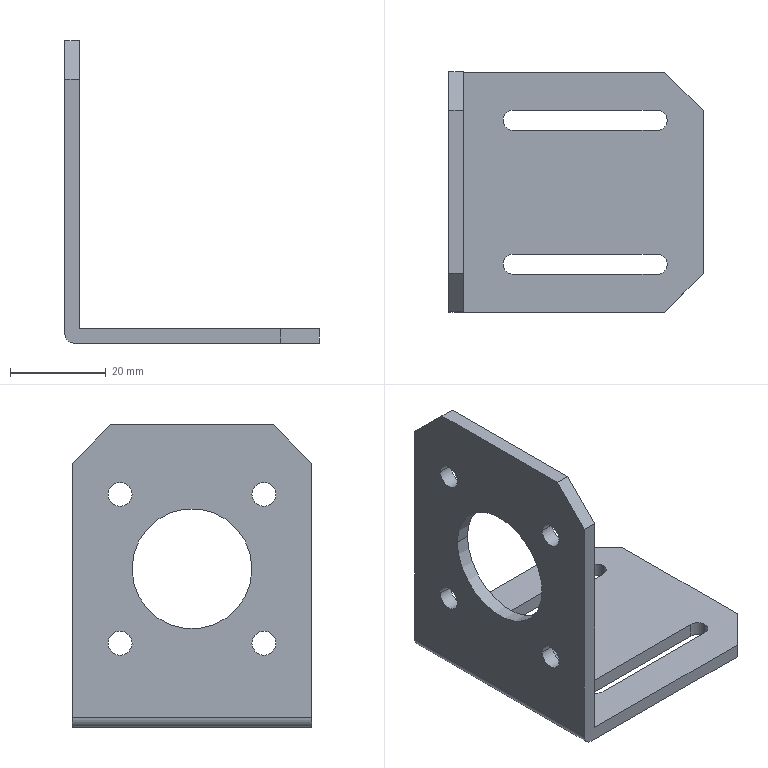Component | SolidWorks | Mount-3 | 1 solid | 33 faces | box 53 x 50 x 63 mm | volume 13976 mm3 | cylinder 17 | plane 16 | commonest cylinder face diameters 5 x8 4.2 x6 25 x2 4 x1
STEP:
#1=COLOUR_RGB('',0.7922,0.8196,0.9333);
#2=FILL_AREA_STYLE_COLOUR('',#1);
#3=FILL_AREA_STYLE('',(#2));
#4=SURFACE_STYLE_FILL_AREA(#3);
#5=SURFACE_SIDE_STYLE('',(#4));
#6=SURFACE_STYLE_USAGE(.BOTH.,#5);
#7=PRESENTATION_STYLE_ASSIGNMENT((#6));
#8=CARTESIAN_POINT('',(-2.678,-2.594,0.1575));
#9=VERTEX_POINT('',#8);
#10=CARTESIAN_POINT('',(-2.595,-2.677,0.1575));
#11=VERTEX_POINT('',#10);
#12=CARTESIAN_POINT('',(-2.678,-2.677,0.1575));
#13=DIRECTION('',(-0.,0.,-1.));
#14=DIRECTION('',(1.,0.,0.));
#15=AXIS2_PLACEMENT_3D('',#12,#13,#14);
#16=CIRCLE('',#15,0.08268);
#17=EDGE_CURVE('',#9,#11,#16,.T.);
#18=ORIENTED_EDGE('',*,*,#17,.T.);
#19=CARTESIAN_POINT('',(-2.595,-2.677,0.2756));
#20=VERTEX_POINT('',#19);
#21=CARTESIAN_POINT('',(-2.595,-2.677,0.1575));
#22=DIRECTION('',(0.,-0.,1.));
#23=VECTOR('',#22,39.37);
#24=LINE('',#21,#23);
#25=EDGE_CURVE('',#11,#20,#24,.T.);
#26=ORIENTED_EDGE('',*,*,#25,.T.);
#27=CARTESIAN_POINT('',(-2.678,-2.594,0.2756));
#28=VERTEX_POINT('',#27);
#29=CARTESIAN_POINT('',(-2.678,-2.677,0.2756));
#30=DIRECTION('',(-0.,0.,-1.));
#31=DIRECTION('',(1.,0.,0.));
#32=AXIS2_PLACEMENT_3D('',#29,#30,#31);
#33=CIRCLE('',#32,0.08268);
#34=EDGE_CURVE('',#28,#20,#33,.T.);
#35=ORIENTED_EDGE('',*,*,#34,.F.);
#36=CARTESIAN_POINT('',(-2.678,-2.594,0.1575));
#37=DIRECTION('',(0.,-0.,1.));
#38=VECTOR('',#37,39.37);
#39=LINE('',#36,#38);
#40=EDGE_CURVE('',#9,#28,#39,.T.);
#41=ORIENTED_EDGE('',*,*,#40,.F.);
#42=EDGE_LOOP('',(#18,#26,#35,#41));
#43=FACE_OUTER_BOUND('',#42,.T.);
#44=CARTESIAN_POINT('',(-2.678,-2.677,0.1575));
#45=DIRECTION('',(0.,-0.,1.));
#46=DIRECTION('',(1.,0.,0.));
#47=AXIS2_PLACEMENT_3D('',#44,#45,#46);
#48=CYLINDRICAL_SURFACE('',#47,0.08268);
#49=ADVANCED_FACE('',(#43),#48,.F.);
#50=CARTESIAN_POINT('',(-2.678,-3.776,0.1575));
#51=VERTEX_POINT('',#50);
#52=CARTESIAN_POINT('',(-2.595,-3.858,0.1575));
#53=VERTEX_POINT('',#52);
#54=CARTESIAN_POINT('',(-2.678,-3.858,0.1575));
#55=DIRECTION('',(-0.,0.,-1.));
#56=DIRECTION('',(-1.,0.,0.));
#57=AXIS2_PLACEMENT_3D('',#54,#55,#56);
#58=CIRCLE('',#57,0.08268);
#59=EDGE_CURVE('',#51,#53,#58,.T.);
#60=ORIENTED_EDGE('',*,*,#59,.T.);
#61=CARTESIAN_POINT('',(-2.595,-3.858,0.2756));
#62=VERTEX_POINT('',#61);
#63=CARTESIAN_POINT('',(-2.595,-3.858,0.1575));
#64=DIRECTION('',(0.,-0.,1.));
#65=VECTOR('',#64,39.37);
#66=LINE('',#63,#65);
#67=EDGE_CURVE('',#53,#62,#66,.T.);
#68=ORIENTED_EDGE('',*,*,#67,.T.);
#69=CARTESIAN_POINT('',(-2.678,-3.776,0.2756));
#70=VERTEX_POINT('',#69);
#71=CARTESIAN_POINT('',(-2.678,-3.858,0.2756));
#72=DIRECTION('',(-0.,0.,-1.));
#73=DIRECTION('',(-1.,0.,0.));
#74=AXIS2_PLACEMENT_3D('',#71,#72,#73);
#75=CIRCLE('',#74,0.08268);
#76=EDGE_CURVE('',#70,#62,#75,.T.);
#77=ORIENTED_EDGE('',*,*,#76,.F.);
#78=CARTESIAN_POINT('',(-2.678,-3.776,0.1575));
#79=DIRECTION('',(0.,-0.,1.));
#80=VECTOR('',#79,39.37);
#81=LINE('',#78,#80);
#82=EDGE_CURVE('',#51,#70,#81,.T.);
#83=ORIENTED_EDGE('',*,*,#82,.F.);
#84=EDGE_LOOP('',(#60,#68,#77,#83));
#85=FACE_OUTER_BOUND('',#84,.T.);
#86=CARTESIAN_POINT('',(-2.678,-3.858,0.1575));
#87=DIRECTION('',(0.,-0.,1.));
#88=DIRECTION('',(1.,0.,0.));
#89=AXIS2_PLACEMENT_3D('',#86,#87,#88);
#90=CYLINDRICAL_SURFACE('',#89,0.08268);
#91=ADVANCED_FACE('',(#85),#90,.F.);
#92=CARTESIAN_POINT('',(-4.268,-3.76,1.457));
#93=VERTEX_POINT('',#92);
#94=CARTESIAN_POINT('',(-4.268,-2.776,1.457));
#95=VERTEX_POINT('',#94);
#96=CARTESIAN_POINT('',(-4.268,-3.268,1.457));
#97=DIRECTION('',(1.,0.,-0.));
#98=DIRECTION('',(-0.,1.,0.));
#99=AXIS2_PLACEMENT_3D('',#96,#97,#98);
#100=CIRCLE('',#99,0.4921);
#101=EDGE_CURVE('',#93,#95,#100,.T.);
#102=ORIENTED_EDGE('',*,*,#101,.T.);
#103=CARTESIAN_POINT('',(-4.387,-2.776,1.457));
#104=VERTEX_POINT('',#103);
#105=CARTESIAN_POINT('',(-4.268,-2.776,1.457));
#106=DIRECTION('',(-1.,-0.,0.));
#107=VECTOR('',#106,39.37);
#108=LINE('',#105,#107);
#109=EDGE_CURVE('',#95,#104,#108,.T.);
#110=ORIENTED_EDGE('',*,*,#109,.T.);
#111=CARTESIAN_POINT('',(-4.387,-3.76,1.457));
#112=VERTEX_POINT('',#111);
#113=CARTESIAN_POINT('',(-4.387,-3.268,1.457));
#114=DIRECTION('',(1.,0.,-0.));
#115=DIRECTION('',(-0.,1.,0.));
#116=AXIS2_PLACEMENT_3D('',#113,#114,#115);
#117=CIRCLE('',#116,0.4921);
#118=EDGE_CURVE('',#112,#104,#117,.T.);
#119=ORIENTED_EDGE('',*,*,#118,.F.);
#120=CARTESIAN_POINT('',(-4.268,-3.76,1.457));
#121=DIRECTION('',(-1.,-0.,0.));
#122=VECTOR('',#121,39.37);
#123=LINE('',#120,#122);
#124=EDGE_CURVE('',#93,#112,#123,.T.);
#125=ORIENTED_EDGE('',*,*,#124,.F.);
#126=EDGE_LOOP('',(#102,#110,#119,#125));
#127=FACE_OUTER_BOUND('',#126,.T.);
#128=CARTESIAN_POINT('',(-4.268,-3.268,1.457));
#129=DIRECTION('',(-1.,-0.,0.));
#130=DIRECTION('',(0.,-1.,0.));
#131=AXIS2_PLACEMENT_3D('',#128,#129,#130);
#132=CYLINDRICAL_SURFACE('',#131,0.4921);
#133=ADVANCED_FACE('',(#127),#132,.F.);
#134=CARTESIAN_POINT('',(-4.268,-3.957,2.067));
#135=VERTEX_POINT('',#134);
#136=CARTESIAN_POINT('',(-4.268,-3.76,2.067));
#137=VERTEX_POINT('',#136);
#138=CARTESIAN_POINT('',(-4.268,-3.858,2.067));
#139=DIRECTION('',(1.,0.,-0.));
#140=DIRECTION('',(0.,-1.,0.));
#141=AXIS2_PLACEMENT_3D('',#138,#139,#140);
#142=CIRCLE('',#141,0.09843);
#143=EDGE_CURVE('',#135,#137,#142,.T.);
#144=ORIENTED_EDGE('',*,*,#143,.T.);
#145=CARTESIAN_POINT('',(-4.387,-3.76,2.067));
#146=VERTEX_POINT('',#145);
#147=CARTESIAN_POINT('',(-4.268,-3.76,2.067));
#148=DIRECTION('',(-1.,-0.,0.));
#149=VECTOR('',#148,39.37);
#150=LINE('',#147,#149);
#151=EDGE_CURVE('',#137,#146,#150,.T.);
#152=ORIENTED_EDGE('',*,*,#151,.T.);
#153=CARTESIAN_POINT('',(-4.387,-3.957,2.067));
#154=VERTEX_POINT('',#153);
#155=CARTESIAN_POINT('',(-4.387,-3.858,2.067));
#156=DIRECTION('',(1.,0.,-0.));
#157=DIRECTION('',(0.,-1.,0.));
#158=AXIS2_PLACEMENT_3D('',#155,#156,#157);
#159=CIRCLE('',#158,0.09843);
#160=EDGE_CURVE('',#154,#146,#159,.T.);
#161=ORIENTED_EDGE('',*,*,#160,.F.);
#162=CARTESIAN_POINT('',(-4.268,-3.957,2.067));
#163=DIRECTION('',(-1.,-0.,0.));
#164=VECTOR('',#163,39.37);
#165=LINE('',#162,#164);
#166=EDGE_CURVE('',#135,#154,#165,.T.);
#167=ORIENTED_EDGE('',*,*,#166,.F.);
#168=EDGE_LOOP('',(#144,#152,#161,#167));
#169=FACE_OUTER_BOUND('',#168,.T.);
#170=CARTESIAN_POINT('',(-4.268,-3.858,2.067));
#171=DIRECTION('',(-1.,-0.,0.));
#172=DIRECTION('',(0.,-1.,0.));
#173=AXIS2_PLACEMENT_3D('',#170,#171,#172);
#174=CYLINDRICAL_SURFACE('',#173,0.09843);
#175=ADVANCED_FACE('',(#169),#174,.F.);
#176=CARTESIAN_POINT('',(-4.268,-2.776,2.067));
#177=VERTEX_POINT('',#176);
#178=CARTESIAN_POINT('',(-4.268,-2.579,2.067));
#179=VERTEX_POINT('',#178);
#180=CARTESIAN_POINT('',(-4.268,-2.677,2.067));
#181=DIRECTION('',(1.,0.,-0.));
#182=DIRECTION('',(0.,1.,0.));
#183=AXIS2_PLACEMENT_3D('',#180,#181,#182);
#184=CIRCLE('',#183,0.09843);
#185=EDGE_CURVE('',#177,#179,#184,.T.);
#186=ORIENTED_EDGE('',*,*,#185,.T.);
#187=CARTESIAN_POINT('',(-4.387,-2.579,2.067));
#188=VERTEX_POINT('',#187);
#189=CARTESIAN_POINT('',(-4.268,-2.579,2.067));
#190=DIRECTION('',(-1.,-0.,0.));
#191=VECTOR('',#190,39.37);
#192=LINE('',#189,#191);
#193=EDGE_CURVE('',#179,#188,#192,.T.);
#194=ORIENTED_EDGE('',*,*,#193,.T.);
#195=CARTESIAN_POINT('',(-4.387,-2.776,2.067));
#196=VERTEX_POINT('',#195);
#197=CARTESIAN_POINT('',(-4.387,-2.677,2.067));
#198=DIRECTION('',(1.,0.,-0.));
#199=DIRECTION('',(0.,1.,0.));
#200=AXIS2_PLACEMENT_3D('',#197,#198,#199);
#201=CIRCLE('',#200,0.09843);
#202=EDGE_CURVE('',#196,#188,#201,.T.);
#203=ORIENTED_EDGE('',*,*,#202,.F.);
#204=CARTESIAN_POINT('',(-4.268,-2.776,2.067));
#205=DIRECTION('',(-1.,-0.,0.));
#206=VECTOR('',#205,39.37);
#207=LINE('',#204,#206);
#208=EDGE_CURVE('',#177,#196,#207,.T.);
#209=ORIENTED_EDGE('',*,*,#208,.F.);
#210=EDGE_LOOP('',(#186,#194,#203,#209));
#211=FACE_OUTER_BOUND('',#210,.T.);
#212=CARTESIAN_POINT('',(-4.268,-2.677,2.067));
#213=DIRECTION('',(-1.,-0.,0.));
#214=DIRECTION('',(0.,-1.,0.));
#215=AXIS2_PLACEMENT_3D('',#212,#213,#214);
#216=CYLINDRICAL_SURFACE('',#215,0.09843);
#217=ADVANCED_FACE('',(#211),#216,.F.);
#218=CARTESIAN_POINT('',(-4.268,-2.776,0.8465));
#219=VERTEX_POINT('',#218);
#220=CARTESIAN_POINT('',(-4.268,-2.579,0.8465));
#221=VERTEX_POINT('',#220);
#222=CARTESIAN_POINT('',(-4.268,-2.677,0.8465));
#223=DIRECTION('',(1.,0.,-0.));
#224=DIRECTION('',(0.,-1.,0.));
#225=AXIS2_PLACEMENT_3D('',#222,#223,#224);
#226=CIRCLE('',#225,0.09843);
#227=EDGE_CURVE('',#219,#221,#226,.T.);
#228=ORIENTED_EDGE('',*,*,#227,.T.);
#229=CARTESIAN_POINT('',(-4.387,-2.579,0.8465));
#230=VERTEX_POINT('',#229);
#231=CARTESIAN_POINT('',(-4.268,-2.579,0.8465));
#232=DIRECTION('',(-1.,-0.,0.));
#233=VECTOR('',#232,39.37);
#234=LINE('',#231,#233);
#235=EDGE_CURVE('',#221,#230,#234,.T.);
#236=ORIENTED_EDGE('',*,*,#235,.T.);
#237=CARTESIAN_POINT('',(-4.387,-2.776,0.8465));
#238=VERTEX_POINT('',#237);
#239=CARTESIAN_POINT('',(-4.387,-2.677,0.8465));
#240=DIRECTION('',(1.,0.,-0.));
#241=DIRECTION('',(0.,-1.,0.));
#242=AXIS2_PLACEMENT_3D('',#239,#240,#241);
#243=CIRCLE('',#242,0.09843);
#244=EDGE_CURVE('',#238,#230,#243,.T.);
#245=ORIENTED_EDGE('',*,*,#244,.F.);
#246=CARTESIAN_POINT('',(-4.268,-2.776,0.8465));
#247=DIRECTION('',(-1.,-0.,0.));
#248=VECTOR('',#247,39.37);
#249=LINE('',#246,#248);
#250=EDGE_CURVE('',#219,#238,#249,.T.);
#251=ORIENTED_EDGE('',*,*,#250,.F.);
#252=EDGE_LOOP('',(#228,#236,#245,#251));
#253=FACE_OUTER_BOUND('',#252,.T.);
#254=CARTESIAN_POINT('',(-4.268,-2.677,0.8465));
#255=DIRECTION('',(-1.,-0.,0.));
#256=DIRECTION('',(0.,-1.,0.));
#257=AXIS2_PLACEMENT_3D('',#254,#255,#256);
#258=CYLINDRICAL_SURFACE('',#257,0.09843);
#259=ADVANCED_FACE('',(#253),#258,.F.);
#260=CARTESIAN_POINT('',(-4.268,-3.957,0.8465));
#261=VERTEX_POINT('',#260);
#262=CARTESIAN_POINT('',(-4.268,-3.76,0.8465));
#263=VERTEX_POINT('',#262);
#264=CARTESIAN_POINT('',(-4.268,-3.858,0.8465));
#265=DIRECTION('',(1.,0.,-0.));
#266=DIRECTION('',(0.,1.,0.));
#267=AXIS2_PLACEMENT_3D('',#264,#265,#266);
#268=CIRCLE('',#267,0.09843);
#269=EDGE_CURVE('',#261,#263,#268,.T.);
#270=ORIENTED_EDGE('',*,*,#269,.T.);
#271=CARTESIAN_POINT('',(-4.387,-3.76,0.8465));
#272=VERTEX_POINT('',#271);
#273=CARTESIAN_POINT('',(-4.268,-3.76,0.8465));
#274=DIRECTION('',(-1.,-0.,0.));
#275=VECTOR('',#274,39.37);
#276=LINE('',#273,#275);
#277=EDGE_CURVE('',#263,#272,#276,.T.);
#278=ORIENTED_EDGE('',*,*,#277,.T.);
#279=CARTESIAN_POINT('',(-4.387,-3.957,0.8465));
#280=VERTEX_POINT('',#279);
#281=CARTESIAN_POINT('',(-4.387,-3.858,0.8465));
#282=DIRECTION('',(1.,0.,-0.));
#283=DIRECTION('',(0.,1.,0.));
#284=AXIS2_PLACEMENT_3D('',#281,#282,#283);
#285=CIRCLE('',#284,0.09843);
#286=EDGE_CURVE('',#280,#272,#285,.T.);
#287=ORIENTED_EDGE('',*,*,#286,.F.);
#288=CARTESIAN_POINT('',(-4.268,-3.957,0.8465));
#289=DIRECTION('',(-1.,-0.,0.));
#290=VECTOR('',#289,39.37);
#291=LINE('',#288,#290);
#292=EDGE_CURVE('',#261,#280,#291,.T.);
#293=ORIENTED_EDGE('',*,*,#292,.F.);
#294=EDGE_LOOP('',(#270,#278,#287,#293));
#295=FACE_OUTER_BOUND('',#294,.T.);
#296=CARTESIAN_POINT('',(-4.268,-3.858,0.8465));
#297=DIRECTION('',(-1.,-0.,0.));
#298=DIRECTION('',(0.,-1.,0.));
#299=AXIS2_PLACEMENT_3D('',#296,#297,#298);
#300=CYLINDRICAL_SURFACE('',#299,0.09843);
#301=ADVANCED_FACE('',(#295),#300,.F.);
#302=CARTESIAN_POINT('',(-4.268,-4.252,2.323));
#303=VERTEX_POINT('',#302);
#304=CARTESIAN_POINT('',(-4.268,-4.252,0.2756));
#305=VERTEX_POINT('',#304);
#306=CARTESIAN_POINT('',(-4.268,-4.252,0.2756));
#307=DIRECTION('',(-0.,0.,-1.));
#308=VECTOR('',#307,39.37);
#309=LINE('',#306,#308);
#310=EDGE_CURVE('',#303,#305,#309,.T.);
#311=ORIENTED_EDGE('',*,*,#310,.T.);
#312=CARTESIAN_POINT('',(-4.268,-2.283,0.2756));
#313=VERTEX_POINT('',#312);
#314=CARTESIAN_POINT('',(-4.268,-4.252,0.2756));
#315=DIRECTION('',(-0.,1.,0.));
#316=VECTOR('',#315,39.37);
#317=LINE('',#314,#316);
#318=EDGE_CURVE('',#305,#313,#317,.T.);
#319=ORIENTED_EDGE('',*,*,#318,.T.);
#320=CARTESIAN_POINT('',(-4.268,-2.283,2.323));
#321=VERTEX_POINT('',#320);
#322=CARTESIAN_POINT('',(-4.268,-2.283,0.2756));
#323=DIRECTION('',(0.,-0.,1.));
#324=VECTOR('',#323,39.37);
#325=LINE('',#322,#324);
#326=EDGE_CURVE('',#313,#321,#325,.T.);
#327=ORIENTED_EDGE('',*,*,#326,.T.);
#328=CARTESIAN_POINT('',(-4.268,-2.598,2.638));
#329=VERTEX_POINT('',#328);
#330=CARTESIAN_POINT('',(-4.268,-2.598,2.638));
#331=DIRECTION('',(0.,-0.7071,0.7071));
#332=VECTOR('',#331,39.37);
#333=LINE('',#330,#332);
#334=EDGE_CURVE('',#321,#329,#333,.T.);
#335=ORIENTED_EDGE('',*,*,#334,.T.);
#336=CARTESIAN_POINT('',(-4.268,-3.937,2.638));
#337=VERTEX_POINT('',#336);
#338=CARTESIAN_POINT('',(-4.268,-3.937,2.638));
#339=DIRECTION('',(0.,-1.,-0.));
#340=VECTOR('',#339,39.37);
#341=LINE('',#338,#340);
#342=EDGE_CURVE('',#329,#337,#341,.T.);
#343=ORIENTED_EDGE('',*,*,#342,.T.);
#344=CARTESIAN_POINT('',(-4.268,-4.252,2.323));
#345=DIRECTION('',(0.,-0.7071,-0.7071));
#346=VECTOR('',#345,39.37);
#347=LINE('',#344,#346);
#348=EDGE_CURVE('',#337,#303,#347,.T.);
#349=ORIENTED_EDGE('',*,*,#348,.T.);
#350=EDGE_LOOP('',(#311,#319,#327,#335,#343,#349));
#351=FACE_OUTER_BOUND('',#350,.T.);
#352=ORIENTED_EDGE('',*,*,#269,.F.);
#353=CARTESIAN_POINT('',(-4.268,-3.858,0.8465));
#354=DIRECTION('',(1.,0.,-0.));
#355=DIRECTION('',(0.,1.,0.));
#356=AXIS2_PLACEMENT_3D('',#353,#354,#355);
#357=CIRCLE('',#356,0.09843);
#358=EDGE_CURVE('',#263,#261,#357,.T.);
#359=ORIENTED_EDGE('',*,*,#358,.F.);
#360=EDGE_LOOP('',(#352,#359));
#361=FACE_BOUND('',#360,.T.);
#362=ORIENTED_EDGE('',*,*,#227,.F.);
#363=CARTESIAN_POINT('',(-4.268,-2.677,0.8465));
#364=DIRECTION('',(1.,0.,-0.));
#365=DIRECTION('',(0.,-1.,0.));
#366=AXIS2_PLACEMENT_3D('',#363,#364,#365);
#367=CIRCLE('',#366,0.09843);
#368=EDGE_CURVE('',#221,#219,#367,.T.);
#369=ORIENTED_EDGE('',*,*,#368,.F.);
#370=EDGE_LOOP('',(#362,#369));
#371=FACE_BOUND('',#370,.T.);
#372=ORIENTED_EDGE('',*,*,#185,.F.);
#373=CARTESIAN_POINT('',(-4.268,-2.677,2.067));
#374=DIRECTION('',(1.,0.,-0.));
#375=DIRECTION('',(0.,1.,0.));
#376=AXIS2_PLACEMENT_3D('',#373,#374,#375);
#377=CIRCLE('',#376,0.09843);
#378=EDGE_CURVE('',#179,#177,#377,.T.);
#379=ORIENTED_EDGE('',*,*,#378,.F.);
#380=EDGE_LOOP('',(#372,#379));
#381=FACE_BOUND('',#380,.T.);
#382=ORIENTED_EDGE('',*,*,#143,.F.);
#383=CARTESIAN_POINT('',(-4.268,-3.858,2.067));
#384=DIRECTION('',(1.,0.,-0.));
#385=DIRECTION('',(0.,-1.,0.));
#386=AXIS2_PLACEMENT_3D('',#383,#384,#385);
#387=CIRCLE('',#386,0.09843);
#388=EDGE_CURVE('',#137,#135,#387,.T.);
#389=ORIENTED_EDGE('',*,*,#388,.F.);
#390=EDGE_LOOP('',(#382,#389));
#391=FACE_BOUND('',#390,.T.);
#392=ORIENTED_EDGE('',*,*,#101,.F.);
#393=CARTESIAN_POINT('',(-4.268,-3.268,1.457));
#394=DIRECTION('',(1.,0.,-0.));
#395=DIRECTION('',(-0.,1.,0.));
#396=AXIS2_PLACEMENT_3D('',#393,#394,#395);
#397=CIRCLE('',#396,0.4921);
#398=EDGE_CURVE('',#95,#93,#397,.T.);
#399=ORIENTED_EDGE('',*,*,#398,.F.);
#400=EDGE_LOOP('',(#392,#399));
#401=FACE_BOUND('',#400,.T.);
#402=CARTESIAN_POINT('',(-4.268,-3.268,1.457));
#403=DIRECTION('',(-1.,-0.,0.));
#404=DIRECTION('',(0.,-1.,-0.));
#405=AXIS2_PLACEMENT_3D('',#402,#403,#404);
#406=PLANE('',#405);
#407=ADVANCED_FACE('',(#351,#361,#371,#381,#391,#401),#406,.F.);
#408=ORIENTED_EDGE('',*,*,#160,.T.);
#409=CARTESIAN_POINT('',(-4.387,-3.858,2.067));
#410=DIRECTION('',(1.,0.,-0.));
#411=DIRECTION('',(0.,-1.,0.));
#412=AXIS2_PLACEMENT_3D('',#409,#410,#411);
#413=CIRCLE('',#412,0.09843);
#414=EDGE_CURVE('',#146,#154,#413,.T.);
#415=ORIENTED_EDGE('',*,*,#414,.T.);
#416=EDGE_LOOP('',(#408,#415));
#417=FACE_BOUND('',#416,.T.);
#418=ORIENTED_EDGE('',*,*,#244,.T.);
#419=CARTESIAN_POINT('',(-4.387,-2.677,0.8465));
#420=DIRECTION('',(1.,0.,-0.));
#421=DIRECTION('',(0.,-1.,0.));
#422=AXIS2_PLACEMENT_3D('',#419,#420,#421);
#423=CIRCLE('',#422,0.09843);
#424=EDGE_CURVE('',#230,#238,#423,.T.);
#425=ORIENTED_EDGE('',*,*,#424,.T.);
#426=EDGE_LOOP('',(#418,#425));
#427=FACE_BOUND('',#426,.T.);
#428=CARTESIAN_POINT('',(-4.387,-2.283,0.2362));
#429=VERTEX_POINT('',#428);
#430=CARTESIAN_POINT('',(-4.387,-2.283,2.323));
#431=VERTEX_POINT('',#430);
#432=CARTESIAN_POINT('',(-4.387,-2.283,0.2756));
#433=DIRECTION('',(0.,-0.,1.));
#434=VECTOR('',#433,39.37);
#435=LINE('',#432,#434);
#436=EDGE_CURVE('',#429,#431,#435,.T.);
#437=ORIENTED_EDGE('',*,*,#436,.F.);
#438=CARTESIAN_POINT('',(-4.387,-4.252,0.2362));
#439=VERTEX_POINT('',#438);
#440=CARTESIAN_POINT('',(-4.387,-4.252,0.2362));
#441=DIRECTION('',(0.,-1.,-0.));
#442=VECTOR('',#441,39.37);
#443=LINE('',#440,#442);
#444=EDGE_CURVE('',#429,#439,#443,.T.);
#445=ORIENTED_EDGE('',*,*,#444,.T.);
#446=CARTESIAN_POINT('',(-4.387,-4.252,2.323));
#447=VERTEX_POINT('',#446);
#448=CARTESIAN_POINT('',(-4.387,-4.252,0.2756));
#449=DIRECTION('',(-0.,0.,-1.));
#450=VECTOR('',#449,39.37);
#451=LINE('',#448,#450);
#452=EDGE_CURVE('',#447,#439,#451,.T.);
#453=ORIENTED_EDGE('',*,*,#452,.F.);
#454=CARTESIAN_POINT('',(-4.387,-3.937,2.638));
#455=VERTEX_POINT('',#454);
#456=CARTESIAN_POINT('',(-4.387,-4.252,2.323));
#457=DIRECTION('',(0.,-0.7071,-0.7071));
#458=VECTOR('',#457,39.37);
#459=LINE('',#456,#458);
#460=EDGE_CURVE('',#455,#447,#459,.T.);
#461=ORIENTED_EDGE('',*,*,#460,.F.);
#462=CARTESIAN_POINT('',(-4.387,-2.598,2.638));
#463=VERTEX_POINT('',#462);
#464=CARTESIAN_POINT('',(-4.387,-3.937,2.638));
#465=DIRECTION('',(0.,-1.,-0.));
#466=VECTOR('',#465,39.37);
#467=LINE('',#464,#466);
#468=EDGE_CURVE('',#463,#455,#467,.T.);
#469=ORIENTED_EDGE('',*,*,#468,.F.);
#470=CARTESIAN_POINT('',(-4.387,-2.598,2.638));
#471=DIRECTION('',(0.,-0.7071,0.7071));
#472=VECTOR('',#471,39.37);
#473=LINE('',#470,#472);
#474=EDGE_CURVE('',#431,#463,#473,.T.);
#475=ORIENTED_EDGE('',*,*,#474,.F.);
#476=EDGE_LOOP('',(#437,#445,#453,#461,#469,#475));
#477=FACE_OUTER_BOUND('',#476,.T.);
#478=ORIENTED_EDGE('',*,*,#286,.T.);
#479=CARTESIAN_POINT('',(-4.387,-3.858,0.8465));
#480=DIRECTION('',(1.,0.,-0.));
#481=DIRECTION('',(0.,1.,0.));
#482=AXIS2_PLACEMENT_3D('',#479,#480,#481);
#483=CIRCLE('',#482,0.09843);
#484=EDGE_CURVE('',#272,#280,#483,.T.);
#485=ORIENTED_EDGE('',*,*,#484,.T.);
#486=EDGE_LOOP('',(#478,#485));
#487=FACE_BOUND('',#486,.T.);
#488=ORIENTED_EDGE('',*,*,#202,.T.);
#489=CARTESIAN_POINT('',(-4.387,-2.677,2.067));
#490=DIRECTION('',(1.,0.,-0.));
#491=DIRECTION('',(0.,1.,0.));
#492=AXIS2_PLACEMENT_3D('',#489,#490,#491);
#493=CIRCLE('',#492,0.09843);
#494=EDGE_CURVE('',#188,#196,#493,.T.);
#495=ORIENTED_EDGE('',*,*,#494,.T.);
#496=EDGE_LOOP('',(#488,#495));
#497=FACE_BOUND('',#496,.T.);
#498=ORIENTED_EDGE('',*,*,#118,.T.);
#499=CARTESIAN_POINT('',(-4.387,-3.268,1.457));
#500=DIRECTION('',(1.,0.,-0.));
#501=DIRECTION('',(-0.,1.,0.));
#502=AXIS2_PLACEMENT_3D('',#499,#500,#501);
#503=CIRCLE('',#502,0.4921);
#504=EDGE_CURVE('',#104,#112,#503,.T.);
#505=ORIENTED_EDGE('',*,*,#504,.T.);
#506=EDGE_LOOP('',(#498,#505));
#507=FACE_BOUND('',#506,.T.);
#508=CARTESIAN_POINT('',(-4.387,-3.268,1.457));
#509=DIRECTION('',(-1.,-0.,0.));
#510=DIRECTION('',(0.,-1.,-0.));
#511=AXIS2_PLACEMENT_3D('',#508,#509,#510);
#512=PLANE('',#511);
#513=ADVANCED_FACE('',(#417,#427,#477,#487,#497,#507),#512,.T.);
#514=ORIENTED_EDGE('',*,*,#452,.T.);
#515=CARTESIAN_POINT('',(-4.308,-4.252,0.1575));
#516=VERTEX_POINT('',#515);
#517=CARTESIAN_POINT('',(-4.308,-4.252,0.2362));
#518=DIRECTION('',(0.,-1.,-0.));
#519=DIRECTION('',(-1.,0.,-0.));
#520=AXIS2_PLACEMENT_3D('',#517,#518,#519);
#521=CIRCLE('',#520,0.07874);
#522=EDGE_CURVE('',#439,#516,#521,.T.);
#523=ORIENTED_EDGE('',*,*,#522,.T.);
#524=CARTESIAN_POINT('',(-2.615,-4.252,0.1575));
#525=VERTEX_POINT('',#524);
#526=CARTESIAN_POINT('',(-4.387,-4.252,0.1575));
#527=DIRECTION('',(-1.,-0.,0.));
#528=VECTOR('',#527,39.37);
#529=LINE('',#526,#528);
#530=EDGE_CURVE('',#525,#516,#529,.T.);
#531=ORIENTED_EDGE('',*,*,#530,.F.);
#532=CARTESIAN_POINT('',(-2.615,-4.252,0.2756));
#533=VERTEX_POINT('',#532);
#534=CARTESIAN_POINT('',(-2.615,-4.252,0.1575));
#535=DIRECTION('',(0.,-0.,1.));
#536=VECTOR('',#535,39.37);
#537=LINE('',#534,#536);
#538=EDGE_CURVE('',#525,#533,#537,.T.);
#539=ORIENTED_EDGE('',*,*,#538,.T.);
#540=CARTESIAN_POINT('',(-4.387,-4.252,0.2756));
#541=DIRECTION('',(-1.,-0.,0.));
#542=VECTOR('',#541,39.37);
#543=LINE('',#540,#542);
#544=EDGE_CURVE('',#533,#305,#543,.T.);
#545=ORIENTED_EDGE('',*,*,#544,.T.);
#546=ORIENTED_EDGE('',*,*,#310,.F.);
#547=CARTESIAN_POINT('',(-4.268,-4.252,2.323));
#548=DIRECTION('',(-1.,-0.,0.));
#549=VECTOR('',#548,39.37);
#550=LINE('',#547,#549);
#551=EDGE_CURVE('',#303,#447,#550,.T.);
#552=ORIENTED_EDGE('',*,*,#551,.T.);
#553=EDGE_LOOP('',(#514,#523,#531,#539,#545,#546,#552));
#554=FACE_OUTER_BOUND('',#553,.T.);
#555=CARTESIAN_POINT('',(-4.268,-4.252,0.2756));
#556=DIRECTION('',(-0.,1.,0.));
#557=DIRECTION('',(-1.,-0.,0.));
#558=AXIS2_PLACEMENT_3D('',#555,#556,#557);
#559=PLANE('',#558);
#560=ADVANCED_FACE('',(#554),#559,.F.);
#561=CARTESIAN_POINT('',(-4.308,-2.283,0.1575));
#562=VERTEX_POINT('',#561);
#563=CARTESIAN_POINT('',(-2.615,-2.283,0.1575));
#564=VERTEX_POINT('',#563);
#565=CARTESIAN_POINT('',(-4.387,-2.283,0.1575));
#566=DIRECTION('',(1.,0.,-0.));
#567=VECTOR('',#566,39.37);
#568=LINE('',#565,#567);
#569=EDGE_CURVE('',#562,#564,#568,.T.);
#570=ORIENTED_EDGE('',*,*,#569,.F.);
#571=CARTESIAN_POINT('',(-4.308,-2.283,0.2362));
#572=DIRECTION('',(-0.,1.,0.));
#573=DIRECTION('',(1.,0.,0.));
#574=AXIS2_PLACEMENT_3D('',#571,#572,#573);
#575=CIRCLE('',#574,0.07874);
#576=EDGE_CURVE('',#562,#429,#575,.T.);
#577=ORIENTED_EDGE('',*,*,#576,.T.);
#578=ORIENTED_EDGE('',*,*,#436,.T.);
#579=CARTESIAN_POINT('',(-4.268,-2.283,2.323));
#580=DIRECTION('',(-1.,-0.,0.));
#581=VECTOR('',#580,39.37);
#582=LINE('',#579,#581);
#583=EDGE_CURVE('',#321,#431,#582,.T.);
#584=ORIENTED_EDGE('',*,*,#583,.F.);
#585=ORIENTED_EDGE('',*,*,#326,.F.);
#586=CARTESIAN_POINT('',(-2.615,-2.283,0.2756));
#587=VERTEX_POINT('',#586);
#588=CARTESIAN_POINT('',(-4.387,-2.283,0.2756));
#589=DIRECTION('',(1.,0.,-0.));
#590=VECTOR('',#589,39.37);
#591=LINE('',#588,#590);
#592=EDGE_CURVE('',#313,#587,#591,.T.);
#593=ORIENTED_EDGE('',*,*,#592,.T.);
#594=CARTESIAN_POINT('',(-2.615,-2.283,0.1575));
#595=DIRECTION('',(0.,-0.,1.));
#596=VECTOR('',#595,39.37);
#597=LINE('',#594,#596);
#598=EDGE_CURVE('',#564,#587,#597,.T.);
#599=ORIENTED_EDGE('',*,*,#598,.F.);
#600=EDGE_LOOP('',(#570,#577,#578,#584,#585,#593,#599));
#601=FACE_OUTER_BOUND('',#600,.T.);
#602=CARTESIAN_POINT('',(-4.268,-2.283,0.2756));
#603=DIRECTION('',(0.,-1.,-0.));
#604=DIRECTION('',(1.,0.,-0.));
#605=AXIS2_PLACEMENT_3D('',#602,#603,#604);
#606=PLANE('',#605);
#607=ADVANCED_FACE('',(#601),#606,.F.);
#608=ORIENTED_EDGE('',*,*,#474,.T.);
#609=CARTESIAN_POINT('',(-4.268,-2.598,2.638));
#610=DIRECTION('',(-1.,-0.,0.));
#611=VECTOR('',#610,39.37);
#612=LINE('',#609,#611);
#613=EDGE_CURVE('',#329,#463,#612,.T.);
#614=ORIENTED_EDGE('',*,*,#613,.F.);
#615=ORIENTED_EDGE('',*,*,#334,.F.);
#616=ORIENTED_EDGE('',*,*,#583,.T.);
#617=EDGE_LOOP('',(#608,#614,#615,#616));
#618=FACE_OUTER_BOUND('',#617,.T.);
#619=CARTESIAN_POINT('',(-4.268,-2.598,2.638));
#620=DIRECTION('',(0.,-0.7071,-0.7071));
#621=DIRECTION('',(-0.,0.7071,-0.7071));
#622=AXIS2_PLACEMENT_3D('',#619,#620,#621);
#623=PLANE('',#622);
#624=ADVANCED_FACE('',(#618),#623,.F.);
#625=ORIENTED_EDGE('',*,*,#468,.T.);
#626=CARTESIAN_POINT('',(-4.268,-3.937,2.638));
#627=DIRECTION('',(-1.,-0.,0.));
#628=VECTOR('',#627,39.37);
#629=LINE('',#626,#628);
#630=EDGE_CURVE('',#337,#455,#629,.T.);
#631=ORIENTED_EDGE('',*,*,#630,.F.);
#632=ORIENTED_EDGE('',*,*,#342,.F.);
#633=ORIENTED_EDGE('',*,*,#613,.T.);
#634=EDGE_LOOP('',(#625,#631,#632,#633));
#635=FACE_OUTER_BOUND('',#634,.T.);
#636=CARTESIAN_POINT('',(-4.268,-3.937,2.638));
#637=DIRECTION('',(-0.,0.,-1.));
#638=DIRECTION('',(-1.,-0.,0.));
#639=AXIS2_PLACEMENT_3D('',#636,#637,#638);
#640=PLANE('',#639);
#641=ADVANCED_FACE('',(#635),#640,.F.);
#642=ORIENTED_EDGE('',*,*,#460,.T.);
#643=ORIENTED_EDGE('',*,*,#551,.F.);
#644=ORIENTED_EDGE('',*,*,#348,.F.);
#645=ORIENTED_EDGE('',*,*,#630,.T.);
#646=EDGE_LOOP('',(#642,#643,#644,#645));
#647=FACE_OUTER_BOUND('',#646,.T.);
#648=CARTESIAN_POINT('',(-4.268,-4.252,2.323));
#649=DIRECTION('',(-0.,0.7071,-0.7071));
#650=DIRECTION('',(-0.,0.7071,0.7071));
#651=AXIS2_PLACEMENT_3D('',#648,#649,#650);
#652=PLANE('',#651);
#653=ADVANCED_FACE('',(#647),#652,.F.);
#654=ORIENTED_EDGE('',*,*,#277,.F.);
#655=ORIENTED_EDGE('',*,*,#358,.T.);
#656=ORIENTED_EDGE('',*,*,#292,.T.);
#657=ORIENTED_EDGE('',*,*,#484,.F.);
#658=EDGE_LOOP('',(#654,#655,#656,#657));
#659=FACE_OUTER_BOUND('',#658,.T.);
#660=CARTESIAN_POINT('',(-4.268,-3.858,0.8465));
#661=DIRECTION('',(-1.,-0.,0.));
#662=DIRECTION('',(0.,-1.,0.));
#663=AXIS2_PLACEMENT_3D('',#660,#661,#662);
#664=CYLINDRICAL_SURFACE('',#663,0.09843);
#665=ADVANCED_FACE('',(#659),#664,.F.);
#666=ORIENTED_EDGE('',*,*,#235,.F.);
#667=ORIENTED_EDGE('',*,*,#368,.T.);
#668=ORIENTED_EDGE('',*,*,#250,.T.);
#669=ORIENTED_EDGE('',*,*,#424,.F.);
#670=EDGE_LOOP('',(#666,#667,#668,#669));
#671=FACE_OUTER_BOUND('',#670,.T.);
#672=CARTESIAN_POINT('',(-4.268,-2.677,0.8465));
#673=DIRECTION('',(-1.,-0.,0.));
#674=DIRECTION('',(0.,-1.,0.));
#675=AXIS2_PLACEMENT_3D('',#672,#673,#674);
#676=CYLINDRICAL_SURFACE('',#675,0.09843);
#677=ADVANCED_FACE('',(#671),#676,.F.);
#678=ORIENTED_EDGE('',*,*,#193,.F.);
#679=ORIENTED_EDGE('',*,*,#378,.T.);
#680=ORIENTED_EDGE('',*,*,#208,.T.);
#681=ORIENTED_EDGE('',*,*,#494,.F.);
#682=EDGE_LOOP('',(#678,#679,#680,#681));
#683=FACE_OUTER_BOUND('',#682,.T.);
#684=CARTESIAN_POINT('',(-4.268,-2.677,2.067));
#685=DIRECTION('',(-1.,-0.,0.));
#686=DIRECTION('',(0.,-1.,0.));
#687=AXIS2_PLACEMENT_3D('',#684,#685,#686);
#688=CYLINDRICAL_SURFACE('',#687,0.09843);
#689=ADVANCED_FACE('',(#683),#688,.F.);
#690=ORIENTED_EDGE('',*,*,#151,.F.);
#691=ORIENTED_EDGE('',*,*,#388,.T.);
#692=ORIENTED_EDGE('',*,*,#166,.T.);
#693=ORIENTED_EDGE('',*,*,#414,.F.);
#694=EDGE_LOOP('',(#690,#691,#692,#693));
#695=FACE_OUTER_BOUND('',#694,.T.);
#696=CARTESIAN_POINT('',(-4.268,-3.858,2.067));
#697=DIRECTION('',(-1.,-0.,0.));
#698=DIRECTION('',(0.,-1.,0.));
#699=AXIS2_PLACEMENT_3D('',#696,#697,#698);
#700=CYLINDRICAL_SURFACE('',#699,0.09843);
#701=ADVANCED_FACE('',(#695),#700,.F.);
#702=ORIENTED_EDGE('',*,*,#109,.F.);
#703=ORIENTED_EDGE('',*,*,#398,.T.);
#704=ORIENTED_EDGE('',*,*,#124,.T.);
#705=ORIENTED_EDGE('',*,*,#504,.F.);
#706=EDGE_LOOP('',(#702,#703,#704,#705));
#707=FACE_OUTER_BOUND('',#706,.T.);
#708=CARTESIAN_POINT('',(-4.268,-3.268,1.457));
#709=DIRECTION('',(-1.,-0.,0.));
#710=DIRECTION('',(0.,-1.,0.));
#711=AXIS2_PLACEMENT_3D('',#708,#709,#710);
#712=CYLINDRICAL_SURFACE('',#711,0.4921);
#713=ADVANCED_FACE('',(#707),#712,.F.);
#714=CARTESIAN_POINT('',(-3.858,-2.594,0.2756));
#715=VERTEX_POINT('',#714);
#716=CARTESIAN_POINT('',(-2.678,-2.594,0.2756));
#717=DIRECTION('',(1.,0.,-0.));
#718=VECTOR('',#717,39.37);
#719=LINE('',#716,#718);
#720=EDGE_CURVE('',#715,#28,#719,.T.);
#721=ORIENTED_EDGE('',*,*,#720,.T.);
#722=ORIENTED_EDGE('',*,*,#34,.T.);
#723=CARTESIAN_POINT('',(-2.678,-2.76,0.2756));
#724=VERTEX_POINT('',#723);
#725=CARTESIAN_POINT('',(-2.678,-2.677,0.2756));
#726=DIRECTION('',(-0.,0.,-1.));
#727=DIRECTION('',(1.,0.,0.));
#728=AXIS2_PLACEMENT_3D('',#725,#726,#727);
#729=CIRCLE('',#728,0.08268);
#730=EDGE_CURVE('',#20,#724,#729,.T.);
#731=ORIENTED_EDGE('',*,*,#730,.T.);
#732=CARTESIAN_POINT('',(-3.858,-2.76,0.2756));
#733=VERTEX_POINT('',#732);
#734=CARTESIAN_POINT('',(-2.678,-2.76,0.2756));
#735=DIRECTION('',(-1.,-0.,0.));
#736=VECTOR('',#735,39.37);
#737=LINE('',#734,#736);
#738=EDGE_CURVE('',#724,#733,#737,.T.);
#739=ORIENTED_EDGE('',*,*,#738,.T.);
#740=CARTESIAN_POINT('',(-3.858,-2.677,0.2756));
#741=DIRECTION('',(-0.,0.,-1.));
#742=DIRECTION('',(1.,0.,0.));
#743=AXIS2_PLACEMENT_3D('',#740,#741,#742);
#744=CIRCLE('',#743,0.08268);
#745=EDGE_CURVE('',#733,#715,#744,.T.);
#746=ORIENTED_EDGE('',*,*,#745,.T.);
#747=EDGE_LOOP('',(#721,#722,#731,#739,#746));
#748=FACE_BOUND('',#747,.T.);
#749=CARTESIAN_POINT('',(-3.858,-3.776,0.2756));
#750=VERTEX_POINT('',#749);
#751=CARTESIAN_POINT('',(-2.678,-3.776,0.2756));
#752=DIRECTION('',(1.,0.,-0.));
#753=VECTOR('',#752,39.37);
#754=LINE('',#751,#753);
#755=EDGE_CURVE('',#750,#70,#754,.T.);
#756=ORIENTED_EDGE('',*,*,#755,.T.);
#757=ORIENTED_EDGE('',*,*,#76,.T.);
#758=CARTESIAN_POINT('',(-2.678,-3.941,0.2756));
#759=VERTEX_POINT('',#758);
#760=CARTESIAN_POINT('',(-2.678,-3.858,0.2756));
#761=DIRECTION('',(-0.,0.,-1.));
#762=DIRECTION('',(-1.,0.,0.));
#763=AXIS2_PLACEMENT_3D('',#760,#761,#762);
#764=CIRCLE('',#763,0.08268);
#765=EDGE_CURVE('',#62,#759,#764,.T.);
#766=ORIENTED_EDGE('',*,*,#765,.T.);
#767=CARTESIAN_POINT('',(-3.858,-3.941,0.2756));
#768=VERTEX_POINT('',#767);
#769=CARTESIAN_POINT('',(-2.678,-3.941,0.2756));
#770=DIRECTION('',(-1.,-0.,0.));
#771=VECTOR('',#770,39.37);
#772=LINE('',#769,#771);
#773=EDGE_CURVE('',#759,#768,#772,.T.);
#774=ORIENTED_EDGE('',*,*,#773,.T.);
#775=CARTESIAN_POINT('',(-3.858,-3.858,0.2756));
#776=DIRECTION('',(-0.,0.,-1.));
#777=DIRECTION('',(-1.,0.,0.));
#778=AXIS2_PLACEMENT_3D('',#775,#776,#777);
#779=CIRCLE('',#778,0.08268);
#780=EDGE_CURVE('',#768,#750,#779,.T.);
#781=ORIENTED_EDGE('',*,*,#780,.T.);
#782=EDGE_LOOP('',(#756,#757,#766,#774,#781));
#783=FACE_BOUND('',#782,.T.);
#784=ORIENTED_EDGE('',*,*,#318,.F.);
#785=ORIENTED_EDGE('',*,*,#544,.F.);
#786=CARTESIAN_POINT('',(-2.3,-3.937,0.2756));
#787=VERTEX_POINT('',#786);
#788=CARTESIAN_POINT('',(-2.615,-4.252,0.2756));
#789=DIRECTION('',(-0.7071,-0.7071,-0.));
#790=VECTOR('',#789,39.37);
#791=LINE('',#788,#790);
#792=EDGE_CURVE('',#787,#533,#791,.T.);
#793=ORIENTED_EDGE('',*,*,#792,.F.);
#794=CARTESIAN_POINT('',(-2.3,-2.598,0.2756));
#795=VERTEX_POINT('',#794);
#796=CARTESIAN_POINT('',(-2.3,-3.937,0.2756));
#797=DIRECTION('',(0.,-1.,-0.));
#798=VECTOR('',#797,39.37);
#799=LINE('',#796,#798);
#800=EDGE_CURVE('',#795,#787,#799,.T.);
#801=ORIENTED_EDGE('',*,*,#800,.F.);
#802=CARTESIAN_POINT('',(-2.3,-2.598,0.2756));
#803=DIRECTION('',(0.7071,-0.7071,-0.));
#804=VECTOR('',#803,39.37);
#805=LINE('',#802,#804);
#806=EDGE_CURVE('',#587,#795,#805,.T.);
#807=ORIENTED_EDGE('',*,*,#806,.F.);
#808=ORIENTED_EDGE('',*,*,#592,.F.);
#809=EDGE_LOOP('',(#784,#785,#793,#801,#807,#808));
#810=FACE_OUTER_BOUND('',#809,.T.);
#811=CARTESIAN_POINT('',(-4.387,-3.268,0.2756));
#812=DIRECTION('',(0.,-0.,1.));
#813=DIRECTION('',(1.,0.,-0.));
#814=AXIS2_PLACEMENT_3D('',#811,#812,#813);
#815=PLANE('',#814);
#816=ADVANCED_FACE('',(#748,#783,#810),#815,.T.);
#817=ORIENTED_EDGE('',*,*,#59,.F.);
#818=CARTESIAN_POINT('',(-3.858,-3.776,0.1575));
#819=VERTEX_POINT('',#818);
#820=CARTESIAN_POINT('',(-2.678,-3.776,0.1575));
#821=DIRECTION('',(1.,0.,-0.));
#822=VECTOR('',#821,39.37);
#823=LINE('',#820,#822);
#824=EDGE_CURVE('',#819,#51,#823,.T.);
#825=ORIENTED_EDGE('',*,*,#824,.F.);
#826=CARTESIAN_POINT('',(-3.858,-3.941,0.1575));
#827=VERTEX_POINT('',#826);
#828=CARTESIAN_POINT('',(-3.858,-3.858,0.1575));
#829=DIRECTION('',(-0.,0.,-1.));
#830=DIRECTION('',(-1.,0.,0.));
#831=AXIS2_PLACEMENT_3D('',#828,#829,#830);
#832=CIRCLE('',#831,0.08268);
#833=EDGE_CURVE('',#827,#819,#832,.T.);
#834=ORIENTED_EDGE('',*,*,#833,.F.);
#835=CARTESIAN_POINT('',(-2.678,-3.941,0.1575));
#836=VERTEX_POINT('',#835);
#837=CARTESIAN_POINT('',(-2.678,-3.941,0.1575));
#838=DIRECTION('',(-1.,-0.,0.));
#839=VECTOR('',#838,39.37);
#840=LINE('',#837,#839);
#841=EDGE_CURVE('',#836,#827,#840,.T.);
#842=ORIENTED_EDGE('',*,*,#841,.F.);
#843=CARTESIAN_POINT('',(-2.678,-3.858,0.1575));
#844=DIRECTION('',(-0.,0.,-1.));
#845=DIRECTION('',(-1.,0.,0.));
#846=AXIS2_PLACEMENT_3D('',#843,#844,#845);
#847=CIRCLE('',#846,0.08268);
#848=EDGE_CURVE('',#53,#836,#847,.T.);
#849=ORIENTED_EDGE('',*,*,#848,.F.);
#850=EDGE_LOOP('',(#817,#825,#834,#842,#849));
#851=FACE_BOUND('',#850,.T.);
#852=ORIENTED_EDGE('',*,*,#530,.T.);
#853=CARTESIAN_POINT('',(-4.308,-2.283,0.1575));
#854=DIRECTION('',(-0.,1.,0.));
#855=VECTOR('',#854,39.37);
#856=LINE('',#853,#855);
#857=EDGE_CURVE('',#516,#562,#856,.T.);
#858=ORIENTED_EDGE('',*,*,#857,.T.);
#859=ORIENTED_EDGE('',*,*,#569,.T.);
#860=CARTESIAN_POINT('',(-2.3,-2.598,0.1575));
#861=VERTEX_POINT('',#860);
#862=CARTESIAN_POINT('',(-2.3,-2.598,0.1575));
#863=DIRECTION('',(0.7071,-0.7071,-0.));
#864=VECTOR('',#863,39.37);
#865=LINE('',#862,#864);
#866=EDGE_CURVE('',#564,#861,#865,.T.);
#867=ORIENTED_EDGE('',*,*,#866,.T.);
#868=CARTESIAN_POINT('',(-2.3,-3.937,0.1575));
#869=VERTEX_POINT('',#868);
#870=CARTESIAN_POINT('',(-2.3,-3.937,0.1575));
#871=DIRECTION('',(0.,-1.,-0.));
#872=VECTOR('',#871,39.37);
#873=LINE('',#870,#872);
#874=EDGE_CURVE('',#861,#869,#873,.T.);
#875=ORIENTED_EDGE('',*,*,#874,.T.);
#876=CARTESIAN_POINT('',(-2.615,-4.252,0.1575));
#877=DIRECTION('',(-0.7071,-0.7071,-0.));
#878=VECTOR('',#877,39.37);
#879=LINE('',#876,#878);
#880=EDGE_CURVE('',#869,#525,#879,.T.);
#881=ORIENTED_EDGE('',*,*,#880,.T.);
#882=EDGE_LOOP('',(#852,#858,#859,#867,#875,#881));
#883=FACE_OUTER_BOUND('',#882,.T.);
#884=ORIENTED_EDGE('',*,*,#17,.F.);
#885=CARTESIAN_POINT('',(-3.858,-2.594,0.1575));
#886=VERTEX_POINT('',#885);
#887=CARTESIAN_POINT('',(-2.678,-2.594,0.1575));
#888=DIRECTION('',(1.,0.,-0.));
#889=VECTOR('',#888,39.37);
#890=LINE('',#887,#889);
#891=EDGE_CURVE('',#886,#9,#890,.T.);
#892=ORIENTED_EDGE('',*,*,#891,.F.);
#893=CARTESIAN_POINT('',(-3.858,-2.76,0.1575));
#894=VERTEX_POINT('',#893);
#895=CARTESIAN_POINT('',(-3.858,-2.677,0.1575));
#896=DIRECTION('',(-0.,0.,-1.));
#897=DIRECTION('',(1.,0.,0.));
#898=AXIS2_PLACEMENT_3D('',#895,#896,#897);
#899=CIRCLE('',#898,0.08268);
#900=EDGE_CURVE('',#894,#886,#899,.T.);
#901=ORIENTED_EDGE('',*,*,#900,.F.);
#902=CARTESIAN_POINT('',(-2.678,-2.76,0.1575));
#903=VERTEX_POINT('',#902);
#904=CARTESIAN_POINT('',(-2.678,-2.76,0.1575));
#905=DIRECTION('',(-1.,-0.,0.));
#906=VECTOR('',#905,39.37);
#907=LINE('',#904,#906);
#908=EDGE_CURVE('',#903,#894,#907,.T.);
#909=ORIENTED_EDGE('',*,*,#908,.F.);
#910=CARTESIAN_POINT('',(-2.678,-2.677,0.1575));
#911=DIRECTION('',(-0.,0.,-1.));
#912=DIRECTION('',(1.,0.,0.));
#913=AXIS2_PLACEMENT_3D('',#910,#911,#912);
#914=CIRCLE('',#913,0.08268);
#915=EDGE_CURVE('',#11,#903,#914,.T.);
#916=ORIENTED_EDGE('',*,*,#915,.F.);
#917=EDGE_LOOP('',(#884,#892,#901,#909,#916));
#918=FACE_BOUND('',#917,.T.);
#919=CARTESIAN_POINT('',(-4.387,-3.268,0.1575));
#920=DIRECTION('',(0.,-0.,1.));
#921=DIRECTION('',(1.,0.,-0.));
#922=AXIS2_PLACEMENT_3D('',#919,#920,#921);
#923=PLANE('',#922);
#924=ADVANCED_FACE('',(#851,#883,#918),#923,.F.);
#925=ORIENTED_EDGE('',*,*,#806,.T.);
#926=CARTESIAN_POINT('',(-2.3,-2.598,0.1575));
#927=DIRECTION('',(0.,-0.,1.));
#928=VECTOR('',#927,39.37);
#929=LINE('',#926,#928);
#930=EDGE_CURVE('',#861,#795,#929,.T.);
#931=ORIENTED_EDGE('',*,*,#930,.F.);
#932=ORIENTED_EDGE('',*,*,#866,.F.);
#933=ORIENTED_EDGE('',*,*,#598,.T.);
#934=EDGE_LOOP('',(#925,#931,#932,#933));
#935=FACE_OUTER_BOUND('',#934,.T.);
#936=CARTESIAN_POINT('',(-2.3,-2.598,0.1575));
#937=DIRECTION('',(-0.7071,-0.7071,-0.));
#938=DIRECTION('',(0.7071,-0.7071,-0.));
#939=AXIS2_PLACEMENT_3D('',#936,#937,#938);
#940=PLANE('',#939);
#941=ADVANCED_FACE('',(#935),#940,.F.);
#942=ORIENTED_EDGE('',*,*,#800,.T.);
#943=CARTESIAN_POINT('',(-2.3,-3.937,0.1575));
#944=DIRECTION('',(0.,-0.,1.));
#945=VECTOR('',#944,39.37);
#946=LINE('',#943,#945);
#947=EDGE_CURVE('',#869,#787,#946,.T.);
#948=ORIENTED_EDGE('',*,*,#947,.F.);
#949=ORIENTED_EDGE('',*,*,#874,.F.);
#950=ORIENTED_EDGE('',*,*,#930,.T.);
#951=EDGE_LOOP('',(#942,#948,#949,#950));
#952=FACE_OUTER_BOUND('',#951,.T.);
#953=CARTESIAN_POINT('',(-2.3,-3.937,0.1575));
#954=DIRECTION('',(-1.,-0.,0.));
#955=DIRECTION('',(0.,-1.,-0.));
#956=AXIS2_PLACEMENT_3D('',#953,#954,#955);
#957=PLANE('',#956);
#958=ADVANCED_FACE('',(#952),#957,.F.);
#959=ORIENTED_EDGE('',*,*,#792,.T.);
#960=ORIENTED_EDGE('',*,*,#538,.F.);
#961=ORIENTED_EDGE('',*,*,#880,.F.);
#962=ORIENTED_EDGE('',*,*,#947,.T.);
#963=EDGE_LOOP('',(#959,#960,#961,#962));
#964=FACE_OUTER_BOUND('',#963,.T.);
#965=CARTESIAN_POINT('',(-2.615,-4.252,0.1575));
#966=DIRECTION('',(-0.7071,0.7071,0.));
#967=DIRECTION('',(-0.7071,-0.7071,-0.));
#968=AXIS2_PLACEMENT_3D('',#965,#966,#967);
#969=PLANE('',#968);
#970=ADVANCED_FACE('',(#964),#969,.F.);
#971=ORIENTED_EDGE('',*,*,#67,.F.);
#972=ORIENTED_EDGE('',*,*,#848,.T.);
#973=CARTESIAN_POINT('',(-2.678,-3.941,0.1575));
#974=DIRECTION('',(0.,-0.,1.));
#975=VECTOR('',#974,39.37);
#976=LINE('',#973,#975);
#977=EDGE_CURVE('',#836,#759,#976,.T.);
#978=ORIENTED_EDGE('',*,*,#977,.T.);
#979=ORIENTED_EDGE('',*,*,#765,.F.);
#980=EDGE_LOOP('',(#971,#972,#978,#979));
#981=FACE_OUTER_BOUND('',#980,.T.);
#982=CARTESIAN_POINT('',(-2.678,-3.858,0.1575));
#983=DIRECTION('',(0.,-0.,1.));
#984=DIRECTION('',(1.,0.,0.));
#985=AXIS2_PLACEMENT_3D('',#982,#983,#984);
#986=CYLINDRICAL_SURFACE('',#985,0.08268);
#987=ADVANCED_FACE('',(#981),#986,.F.);
#988=ORIENTED_EDGE('',*,*,#773,.F.);
#989=ORIENTED_EDGE('',*,*,#977,.F.);
#990=ORIENTED_EDGE('',*,*,#841,.T.);
#991=CARTESIAN_POINT('',(-3.858,-3.941,0.1575));
#992=DIRECTION('',(0.,-0.,1.));
#993=VECTOR('',#992,39.37);
#994=LINE('',#991,#993);
#995=EDGE_CURVE('',#827,#768,#994,.T.);
#996=ORIENTED_EDGE('',*,*,#995,.T.);
#997=EDGE_LOOP('',(#988,#989,#990,#996));
#998=FACE_OUTER_BOUND('',#997,.T.);
#999=CARTESIAN_POINT('',(-2.678,-3.941,0.1575));
#1000=DIRECTION('',(-0.,1.,0.));
#1001=DIRECTION('',(-1.,-0.,0.));
#1002=AXIS2_PLACEMENT_3D('',#999,#1000,#1001);
#1003=PLANE('',#1002);
#1004=ADVANCED_FACE('',(#998),#1003,.T.);
#1005=ORIENTED_EDGE('',*,*,#780,.F.);
#1006=ORIENTED_EDGE('',*,*,#995,.F.);
#1007=ORIENTED_EDGE('',*,*,#833,.T.);
#1008=CARTESIAN_POINT('',(-3.858,-3.776,0.1575));
#1009=DIRECTION('',(0.,-0.,1.));
#1010=VECTOR('',#1009,39.37);
#1011=LINE('',#1008,#1010);
#1012=EDGE_CURVE('',#819,#750,#1011,.T.);
#1013=ORIENTED_EDGE('',*,*,#1012,.T.);
#1014=EDGE_LOOP('',(#1005,#1006,#1007,#1013));
#1015=FACE_OUTER_BOUND('',#1014,.T.);
#1016=CARTESIAN_POINT('',(-3.858,-3.858,0.1575));
#1017=DIRECTION('',(0.,-0.,1.));
#1018=DIRECTION('',(1.,0.,0.));
#1019=AXIS2_PLACEMENT_3D('',#1016,#1017,#1018);
#1020=CYLINDRICAL_SURFACE('',#1019,0.08268);
#1021=ADVANCED_FACE('',(#1015),#1020,.F.);
#1022=ORIENTED_EDGE('',*,*,#755,.F.);
#1023=ORIENTED_EDGE('',*,*,#1012,.F.);
#1024=ORIENTED_EDGE('',*,*,#824,.T.);
#1025=ORIENTED_EDGE('',*,*,#82,.T.);
#1026=EDGE_LOOP('',(#1022,#1023,#1024,#1025));
#1027=FACE_OUTER_BOUND('',#1026,.T.);
#1028=CARTESIAN_POINT('',(-2.678,-3.776,0.1575));
#1029=DIRECTION('',(0.,-1.,-0.));
#1030=DIRECTION('',(1.,0.,-0.));
#1031=AXIS2_PLACEMENT_3D('',#1028,#1029,#1030);
#1032=PLANE('',#1031);
#1033=ADVANCED_FACE('',(#1027),#1032,.T.);
#1034=ORIENTED_EDGE('',*,*,#25,.F.);
#1035=ORIENTED_EDGE('',*,*,#915,.T.);
#1036=CARTESIAN_POINT('',(-2.678,-2.76,0.1575));
#1037=DIRECTION('',(0.,-0.,1.));
#1038=VECTOR('',#1037,39.37);
#1039=LINE('',#1036,#1038);
#1040=EDGE_CURVE('',#903,#724,#1039,.T.);
#1041=ORIENTED_EDGE('',*,*,#1040,.T.);
#1042=ORIENTED_EDGE('',*,*,#730,.F.);
#1043=EDGE_LOOP('',(#1034,#1035,#1041,#1042));
#1044=FACE_OUTER_BOUND('',#1043,.T.);
#1045=CARTESIAN_POINT('',(-2.678,-2.677,0.1575));
#1046=DIRECTION('',(0.,-0.,1.));
#1047=DIRECTION('',(1.,0.,0.));
#1048=AXIS2_PLACEMENT_3D('',#1045,#1046,#1047);
#1049=CYLINDRICAL_SURFACE('',#1048,0.08268);
#1050=ADVANCED_FACE('',(#1044),#1049,.F.);
#1051=ORIENTED_EDGE('',*,*,#738,.F.);
#1052=ORIENTED_EDGE('',*,*,#1040,.F.);
#1053=ORIENTED_EDGE('',*,*,#908,.T.);
#1054=CARTESIAN_POINT('',(-3.858,-2.76,0.1575));
#1055=DIRECTION('',(0.,-0.,1.));
#1056=VECTOR('',#1055,39.37);
#1057=LINE('',#1054,#1056);
#1058=EDGE_CURVE('',#894,#733,#1057,.T.);
#1059=ORIENTED_EDGE('',*,*,#1058,.T.);
#1060=EDGE_LOOP('',(#1051,#1052,#1053,#1059));
#1061=FACE_OUTER_BOUND('',#1060,.T.);
#1062=CARTESIAN_POINT('',(-2.678,-2.76,0.1575));
#1063=DIRECTION('',(-0.,1.,0.));
#1064=DIRECTION('',(-1.,-0.,0.));
#1065=AXIS2_PLACEMENT_3D('',#1062,#1063,#1064);
#1066=PLANE('',#1065);
#1067=ADVANCED_FACE('',(#1061),#1066,.T.);
#1068=ORIENTED_EDGE('',*,*,#745,.F.);
#1069=ORIENTED_EDGE('',*,*,#1058,.F.);
#1070=ORIENTED_EDGE('',*,*,#900,.T.);
#1071=CARTESIAN_POINT('',(-3.858,-2.594,0.1575));
#1072=DIRECTION('',(0.,-0.,1.));
#1073=VECTOR('',#1072,39.37);
#1074=LINE('',#1071,#1073);
#1075=EDGE_CURVE('',#886,#715,#1074,.T.);
#1076=ORIENTED_EDGE('',*,*,#1075,.T.);
#1077=EDGE_LOOP('',(#1068,#1069,#1070,#1076));
#1078=FACE_OUTER_BOUND('',#1077,.T.);
#1079=CARTESIAN_POINT('',(-3.858,-2.677,0.1575));
#1080=DIRECTION('',(0.,-0.,1.));
#1081=DIRECTION('',(1.,0.,0.));
#1082=AXIS2_PLACEMENT_3D('',#1079,#1080,#1081);
#1083=CYLINDRICAL_SURFACE('',#1082,0.08268);
#1084=ADVANCED_FACE('',(#1078),#1083,.F.);
#1085=ORIENTED_EDGE('',*,*,#720,.F.);
#1086=ORIENTED_EDGE('',*,*,#1075,.F.);
#1087=ORIENTED_EDGE('',*,*,#891,.T.);
#1088=ORIENTED_EDGE('',*,*,#40,.T.);
#1089=EDGE_LOOP('',(#1085,#1086,#1087,#1088));
#1090=FACE_OUTER_BOUND('',#1089,.T.);
#1091=CARTESIAN_POINT('',(-2.678,-2.594,0.1575));
#1092=DIRECTION('',(0.,-1.,-0.));
#1093=DIRECTION('',(1.,0.,-0.));
#1094=AXIS2_PLACEMENT_3D('',#1091,#1092,#1093);
#1095=PLANE('',#1094);
#1096=ADVANCED_FACE('',(#1090),#1095,.T.);
#1097=ORIENTED_EDGE('',*,*,#522,.F.);
#1098=ORIENTED_EDGE('',*,*,#444,.F.);
#1099=ORIENTED_EDGE('',*,*,#576,.F.);
#1100=ORIENTED_EDGE('',*,*,#857,.F.);
#1101=EDGE_LOOP('',(#1097,#1098,#1099,#1100));
#1102=FACE_OUTER_BOUND('',#1101,.T.);
#1103=CARTESIAN_POINT('',(-4.308,-3.268,0.2362));
#1104=DIRECTION('',(0.,-1.,-0.));
#1105=DIRECTION('',(1.,0.,0.));
#1106=AXIS2_PLACEMENT_3D('',#1103,#1104,#1105);
#1107=CYLINDRICAL_SURFACE('',#1106,0.07874);
#1108=ADVANCED_FACE('',(#1102),#1107,.T.);
#1109=CLOSED_SHELL('',(#49,#91,#133,#175,#217,#259,#301,#407,#513,#560,#607,#624,#641,#653,#665,#677,#689,#701,#713,#816,#924,#941,#958,#970,#987,#1004,#1021,#1033,#1050,#1067,#1084,#1096,#1108));
#1110=MANIFOLD_SOLID_BREP('',#1109);
#1111=STYLED_ITEM('',(#7),#1110);
#1112=PRESENTATION_LAYER_ASSIGNMENT('','',(#1111));
#1113=(LENGTH_UNIT()NAMED_UNIT(*)SI_UNIT($,.METRE.));
#1114=LENGTH_MEASURE_WITH_UNIT(LENGTH_MEASURE(0.0254),#1113);
#1115=DIMENSIONAL_EXPONENTS(1.,0.,0.,0.,0.,0.,0.);
#1116=(CONVERSION_BASED_UNIT('',#1114)LENGTH_UNIT()NAMED_UNIT(#1115));
#1117=UNCERTAINTY_MEASURE_WITH_UNIT(LENGTH_MEASURE(0.00001),#1116,'','');
#1118=(NAMED_UNIT(*)PLANE_ANGLE_UNIT()SI_UNIT($,.RADIAN.));
#1119=(NAMED_UNIT(*)SI_UNIT($,.STERADIAN.)SOLID_ANGLE_UNIT());
#1120=(GEOMETRIC_REPRESENTATION_CONTEXT(3)GLOBAL_UNCERTAINTY_ASSIGNED_CONTEXT((#1117))GLOBAL_UNIT_ASSIGNED_CONTEXT((#1116,#1118,#1119))REPRESENTATION_CONTEXT('',''));
#1121=MECHANICAL_DESIGN_GEOMETRIC_PRESENTATION_REPRESENTATION('',(#1111),#1120);
#1122=CARTESIAN_POINT('',(0.,0.,0.));
#1123=DIRECTION('',(0.,0.,1.));
#1124=DIRECTION('',(1.,0.,0.));
#1125=AXIS2_PLACEMENT_3D('',#1122,#1123,#1124);
#1126=(LENGTH_UNIT()NAMED_UNIT(*)SI_UNIT($,.METRE.));
#1127=LENGTH_MEASURE_WITH_UNIT(LENGTH_MEASURE(0.0254),#1126);
#1128=DIMENSIONAL_EXPONENTS(1.,0.,0.,0.,0.,0.,0.);
#1129=(CONVERSION_BASED_UNIT('',#1127)LENGTH_UNIT()NAMED_UNIT(#1128));
#1130=UNCERTAINTY_MEASURE_WITH_UNIT(LENGTH_MEASURE(0.00001),#1129,'','');
#1131=(NAMED_UNIT(*)PLANE_ANGLE_UNIT()SI_UNIT($,.RADIAN.));
#1132=(NAMED_UNIT(*)SI_UNIT($,.STERADIAN.)SOLID_ANGLE_UNIT());
#1133=(GEOMETRIC_REPRESENTATION_CONTEXT(3)GLOBAL_UNCERTAINTY_ASSIGNED_CONTEXT((#1130))GLOBAL_UNIT_ASSIGNED_CONTEXT((#1129,#1131,#1132))REPRESENTATION_CONTEXT('',''));
#1134=ADVANCED_BREP_SHAPE_REPRESENTATION('',(#1110,#1125),#1133);